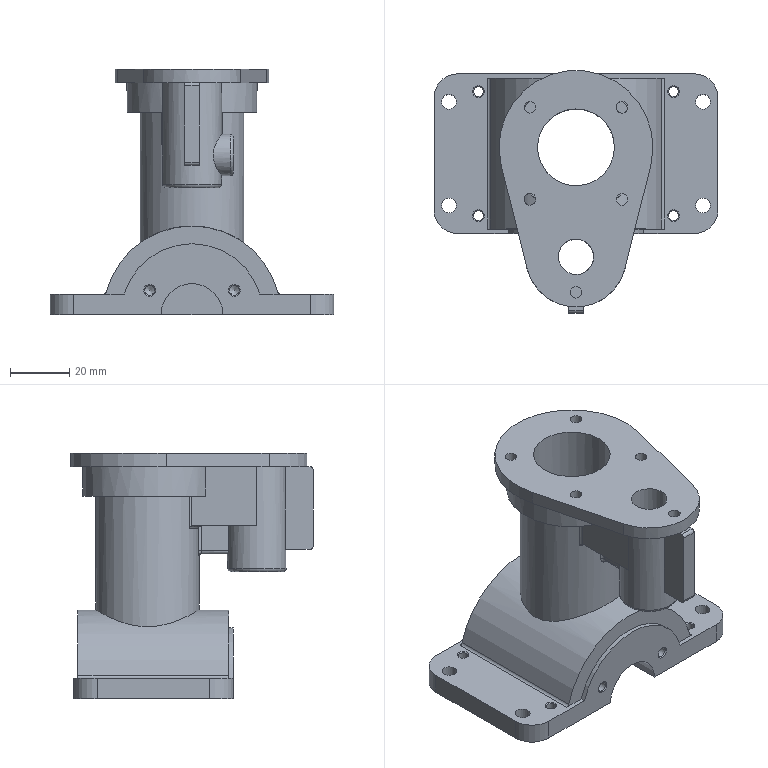Component | NX | ENGINE_BODY | 1 solid | 97 faces | volume 102101 mm3 | cylinder 44 | plane 35 | cone 12 | torus 4 | spline 2 | commonest cylinder face diameters 2 x10 3.3 x6 5 x5 4 x5 16 x4 8 x2 12 x1 26 x1